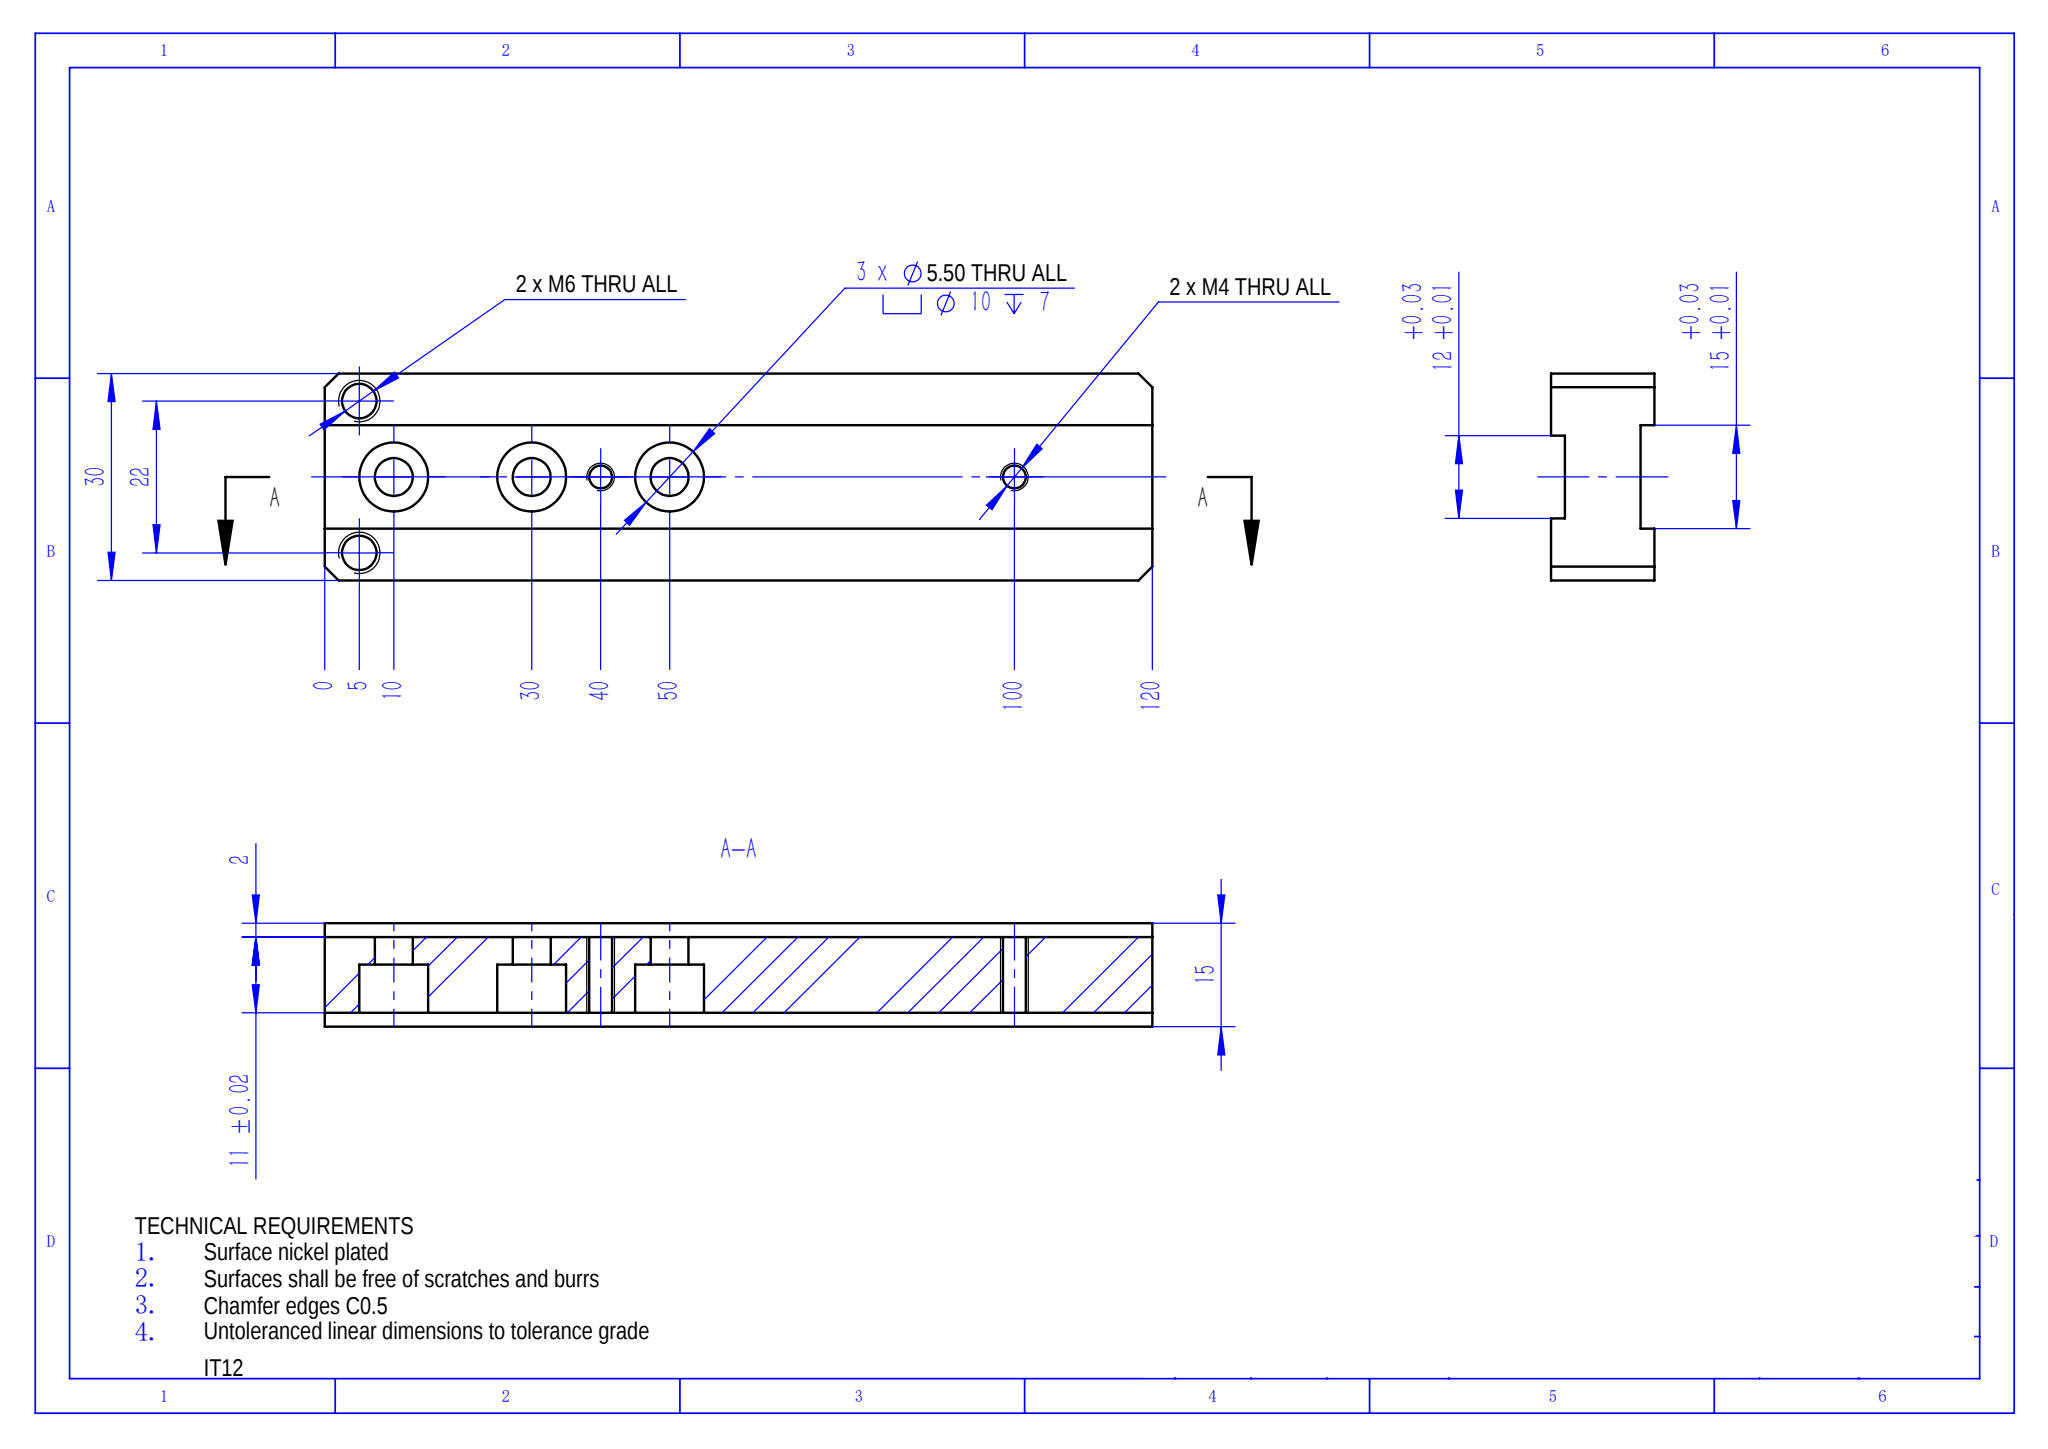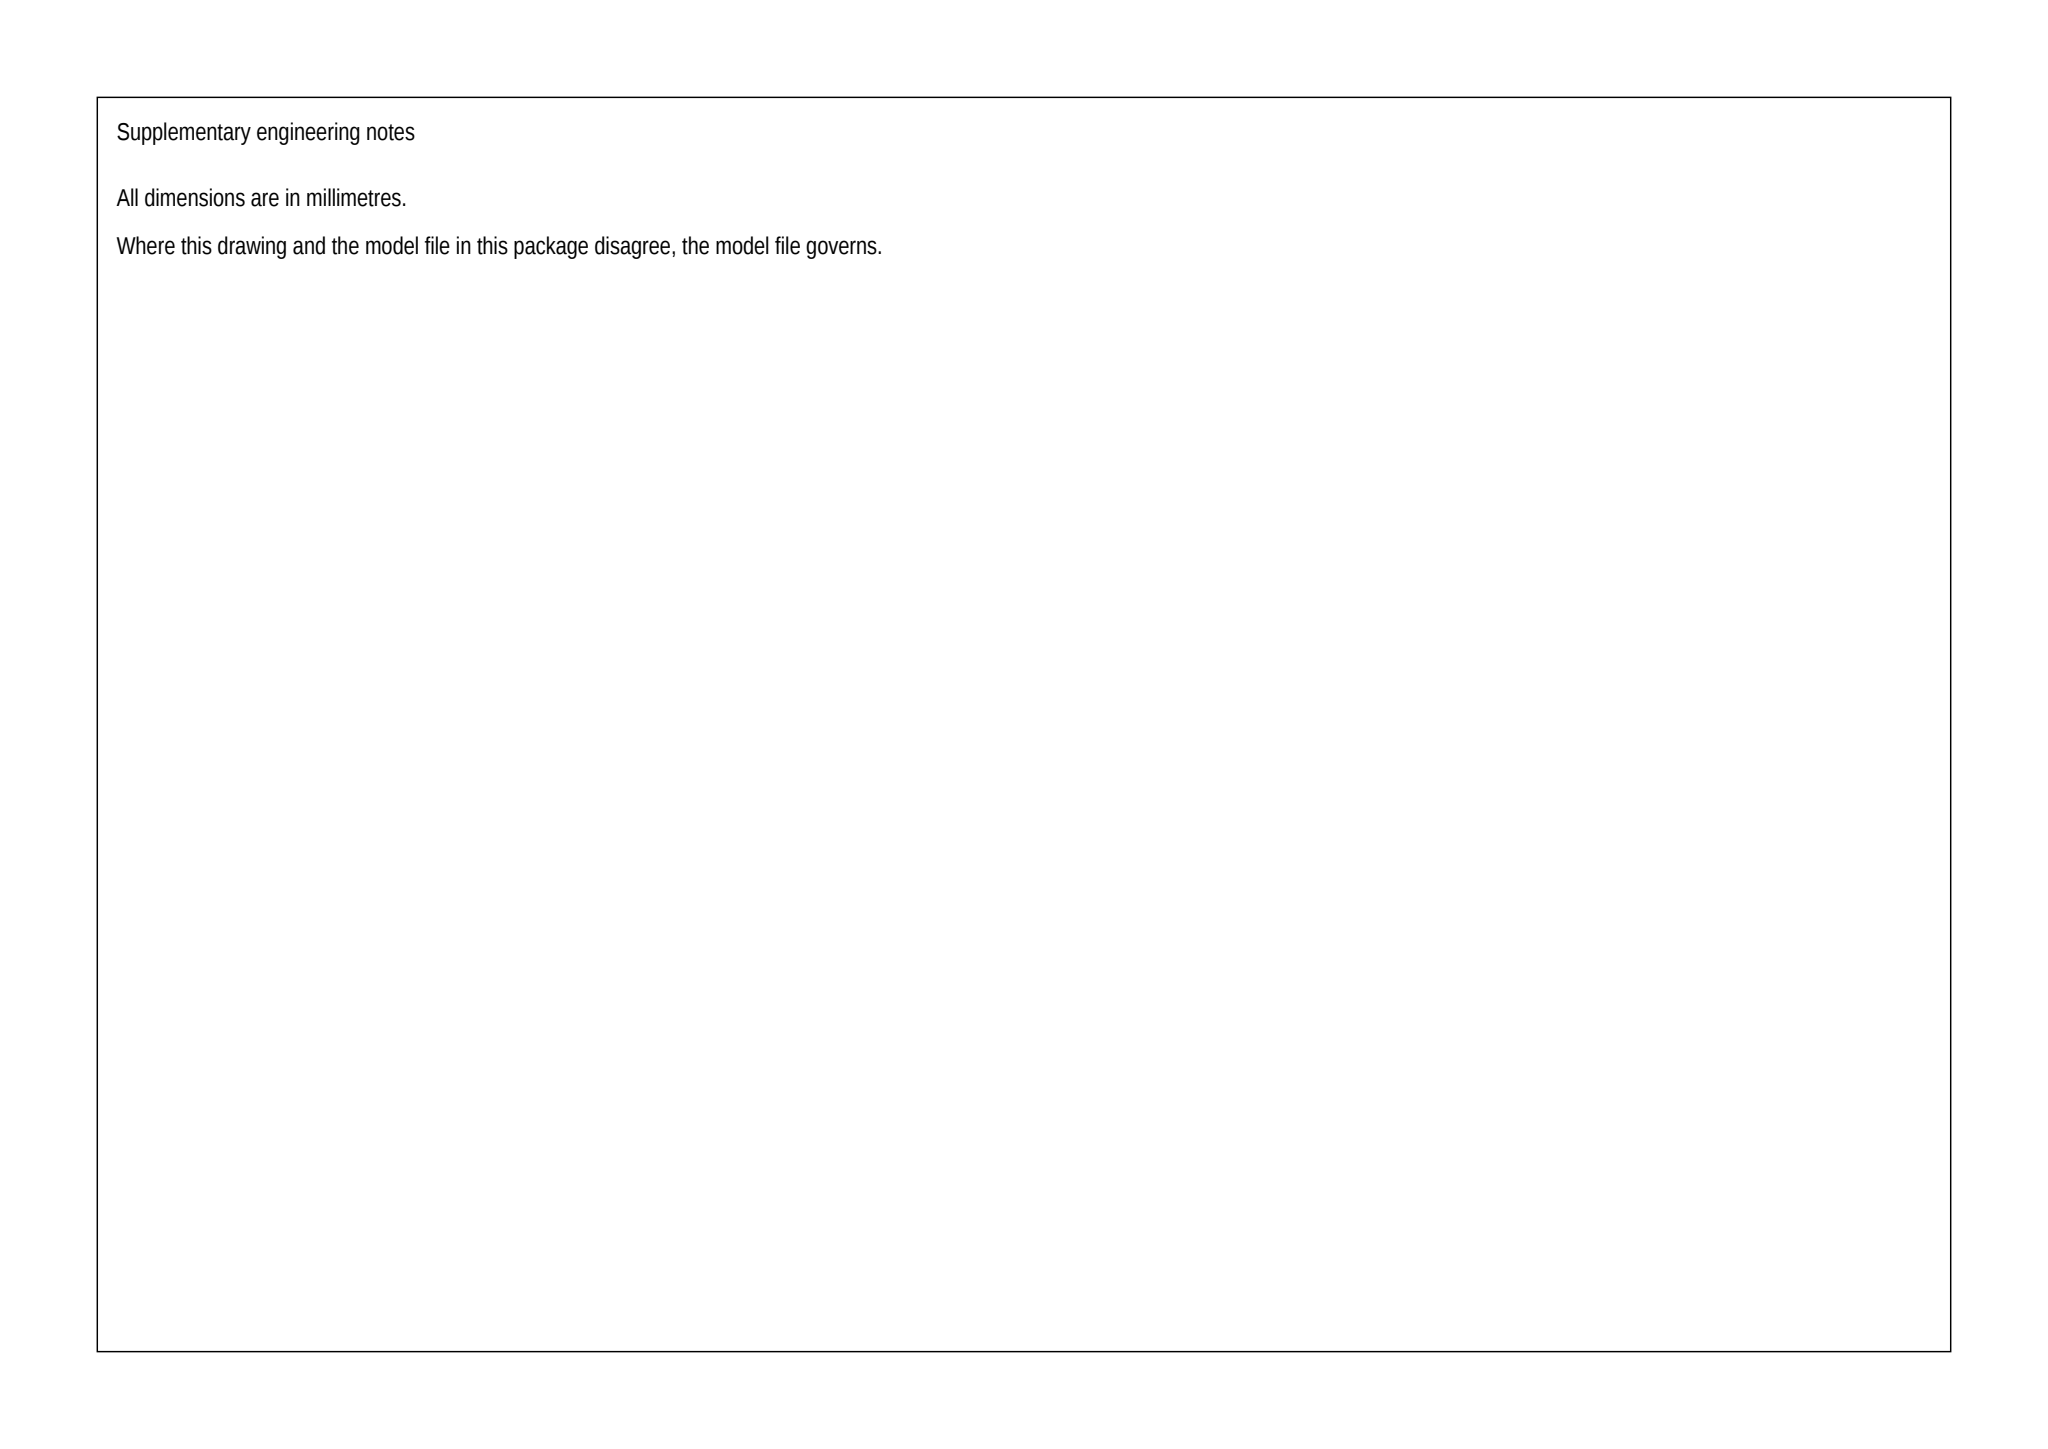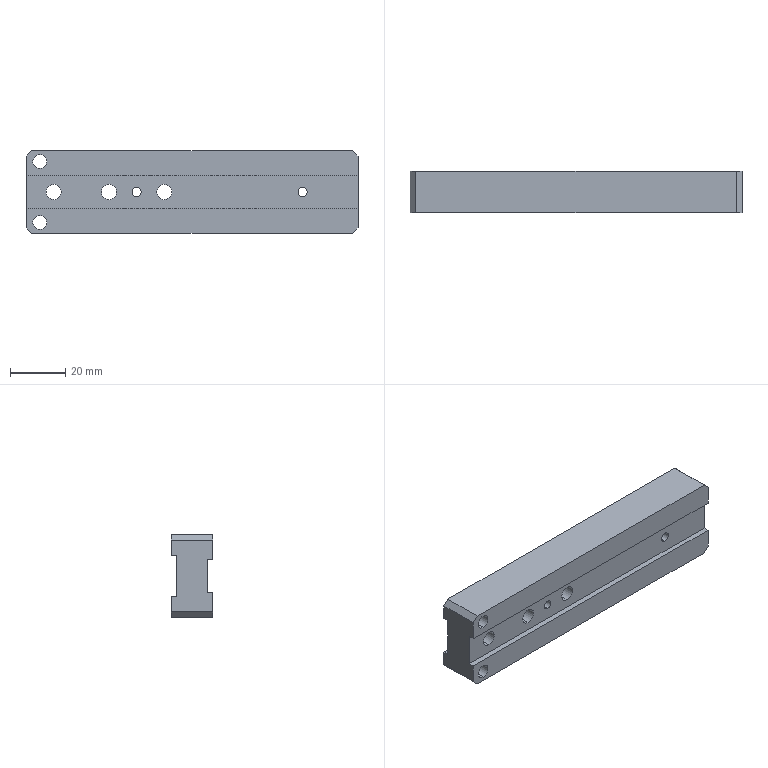Part | SolidWorks | mm | 1 solid | 41 faces | box 120 x 15 x 30 mm | volume 44688 mm3 | plane 21 | cylinder 20 | commonest cylinder face diameters 10 x6 5.5 x6 5 x4 3.3 x4
Drawing notes:
4X C2 CHAMFER AT PLATE CORNERS (SUPERSEDES NOTE 3) | from the solid: 120x15x30 bbox plate with 4 corner chamfers in plan view (X0/X120 end faces vs Z0/Z30 side faces); chamfer legs 2 mm, i.e. corner cut from (0,2) to (2,0) clear of M6 pilot Ø5 at X5, Z4/Z26
build123d program:
from build123d import *

# Parameters (mm, degrees)
SKETCH1_W                                         = 120
SKETCH1_H                                         = 30
BOSS_EXTRUDE1_DEPTH                               = 15
CUT_EXTRUDE3_DEPTH                                = 2
HOLE_SIZE_ACCORDING_TO_HEXAGON_SOCKET_D           = 5.5
HOLE_SIZE_ACCORDING_TO_HEXAGON_SOCKET_CBORE_D     = 10
HOLE_SIZE_ACCORDING_TO_HEXAGON_SOCKET_CBORE_DEPTH = 7
M4_TAPPED_HOLE1_D                                 = 3.3
CUT_EXTRUDE1_DEPTH                                = 2
M6_TAPPED_HOLE1_D                                 = 5
CHAMFER1_SIZE                                     = 2


with BuildPart() as part:
    # Sketch1 → Boss-Extrude1 (new body)
    with BuildSketch(Plane(origin=(0, 0, 0), x_dir=(1, 0, 0), z_dir=(0, 1, 0))):
        with Locations((-60, 0)):
            Rectangle(SKETCH1_W, SKETCH1_H)
    extrude(amount=BOSS_EXTRUDE1_DEPTH)

    # Sketch12 → Cut-Extrude3 (cut)
    with BuildSketch(Plane(origin=(0, 15, 0), x_dir=(1, 0, 0), z_dir=(0, 1, 0))):
        with BuildLine():
            Line((0, 7.5), (-120, 7.5))
            ThreePointArc((-120, 7.5), (-122.121, 6.621), (-123, 4.5))
            Line((-123, 4.5), (-123, -4.5))
            ThreePointArc((-123, -4.5), (-122.121, -6.621), (-120, -7.5))
            Line((-120, -7.5), (0, -7.5))
            Line((0, -7.5), (0, 7.5))
        make_face()
    extrude(amount=-CUT_EXTRUDE3_DEPTH, mode=Mode.SUBTRACT)

    # Hole Size _ according to_ Hexagon Socket (through all)
    with Locations(Plane(origin=(0, 13, 0), x_dir=(1, 0, 0), z_dir=(0, 1, 0))):
        with Locations((-70, 0), (-90, 0), (-110, 0)):
            CounterBoreHole(HOLE_SIZE_ACCORDING_TO_HEXAGON_SOCKET_D / 2, HOLE_SIZE_ACCORDING_TO_HEXAGON_SOCKET_CBORE_D / 2, HOLE_SIZE_ACCORDING_TO_HEXAGON_SOCKET_CBORE_DEPTH)

    # M4 Tapped Hole1 (through all)
    with Locations(Plane(origin=(0, 15, 0), x_dir=(1, 0, 0), z_dir=(0, 1, 0))):
        with Locations((-20, 0), (-80, 0)):
            Hole(M4_TAPPED_HOLE1_D / 2)

    # Sketch8 → Cut-Extrude1 (cut)
    with BuildSketch(Plane.XZ):
        with BuildLine():
            Line((0, 6), (-120, 6))
            ThreePointArc((-120, 6), (-122.121, 5.121), (-123, 3))
            Line((-123, 3), (-123, -3))
            ThreePointArc((-123, -3), (-122.121, -5.121), (-120, -6))
            Line((-120, -6), (0, -6))
            Line((0, -6), (0, 6))
        make_face()
    extrude(amount=-CUT_EXTRUDE1_DEPTH, mode=Mode.SUBTRACT)

    # M6 Tapped Hole1 (through all)
    with Locations(Plane(origin=(0, 15, 0), x_dir=(1, 0, 0), z_dir=(0, 1, 0))):
        with Locations((-115, 11), (-115, -11)):
            Hole(M6_TAPPED_HOLE1_D / 2)

    # Chamfer1
    chamfer1_edges = [part.edges().sort_by_distance(p)[0] for p in [
        (0, 7.5, 15),
        (-120, 7.5, 15),
        (-120, 7.5, -15),
        (0, 7.5, -15),
    ]]
    chamfer(chamfer1_edges, length=CHAMFER1_SIZE)


solid = part.part